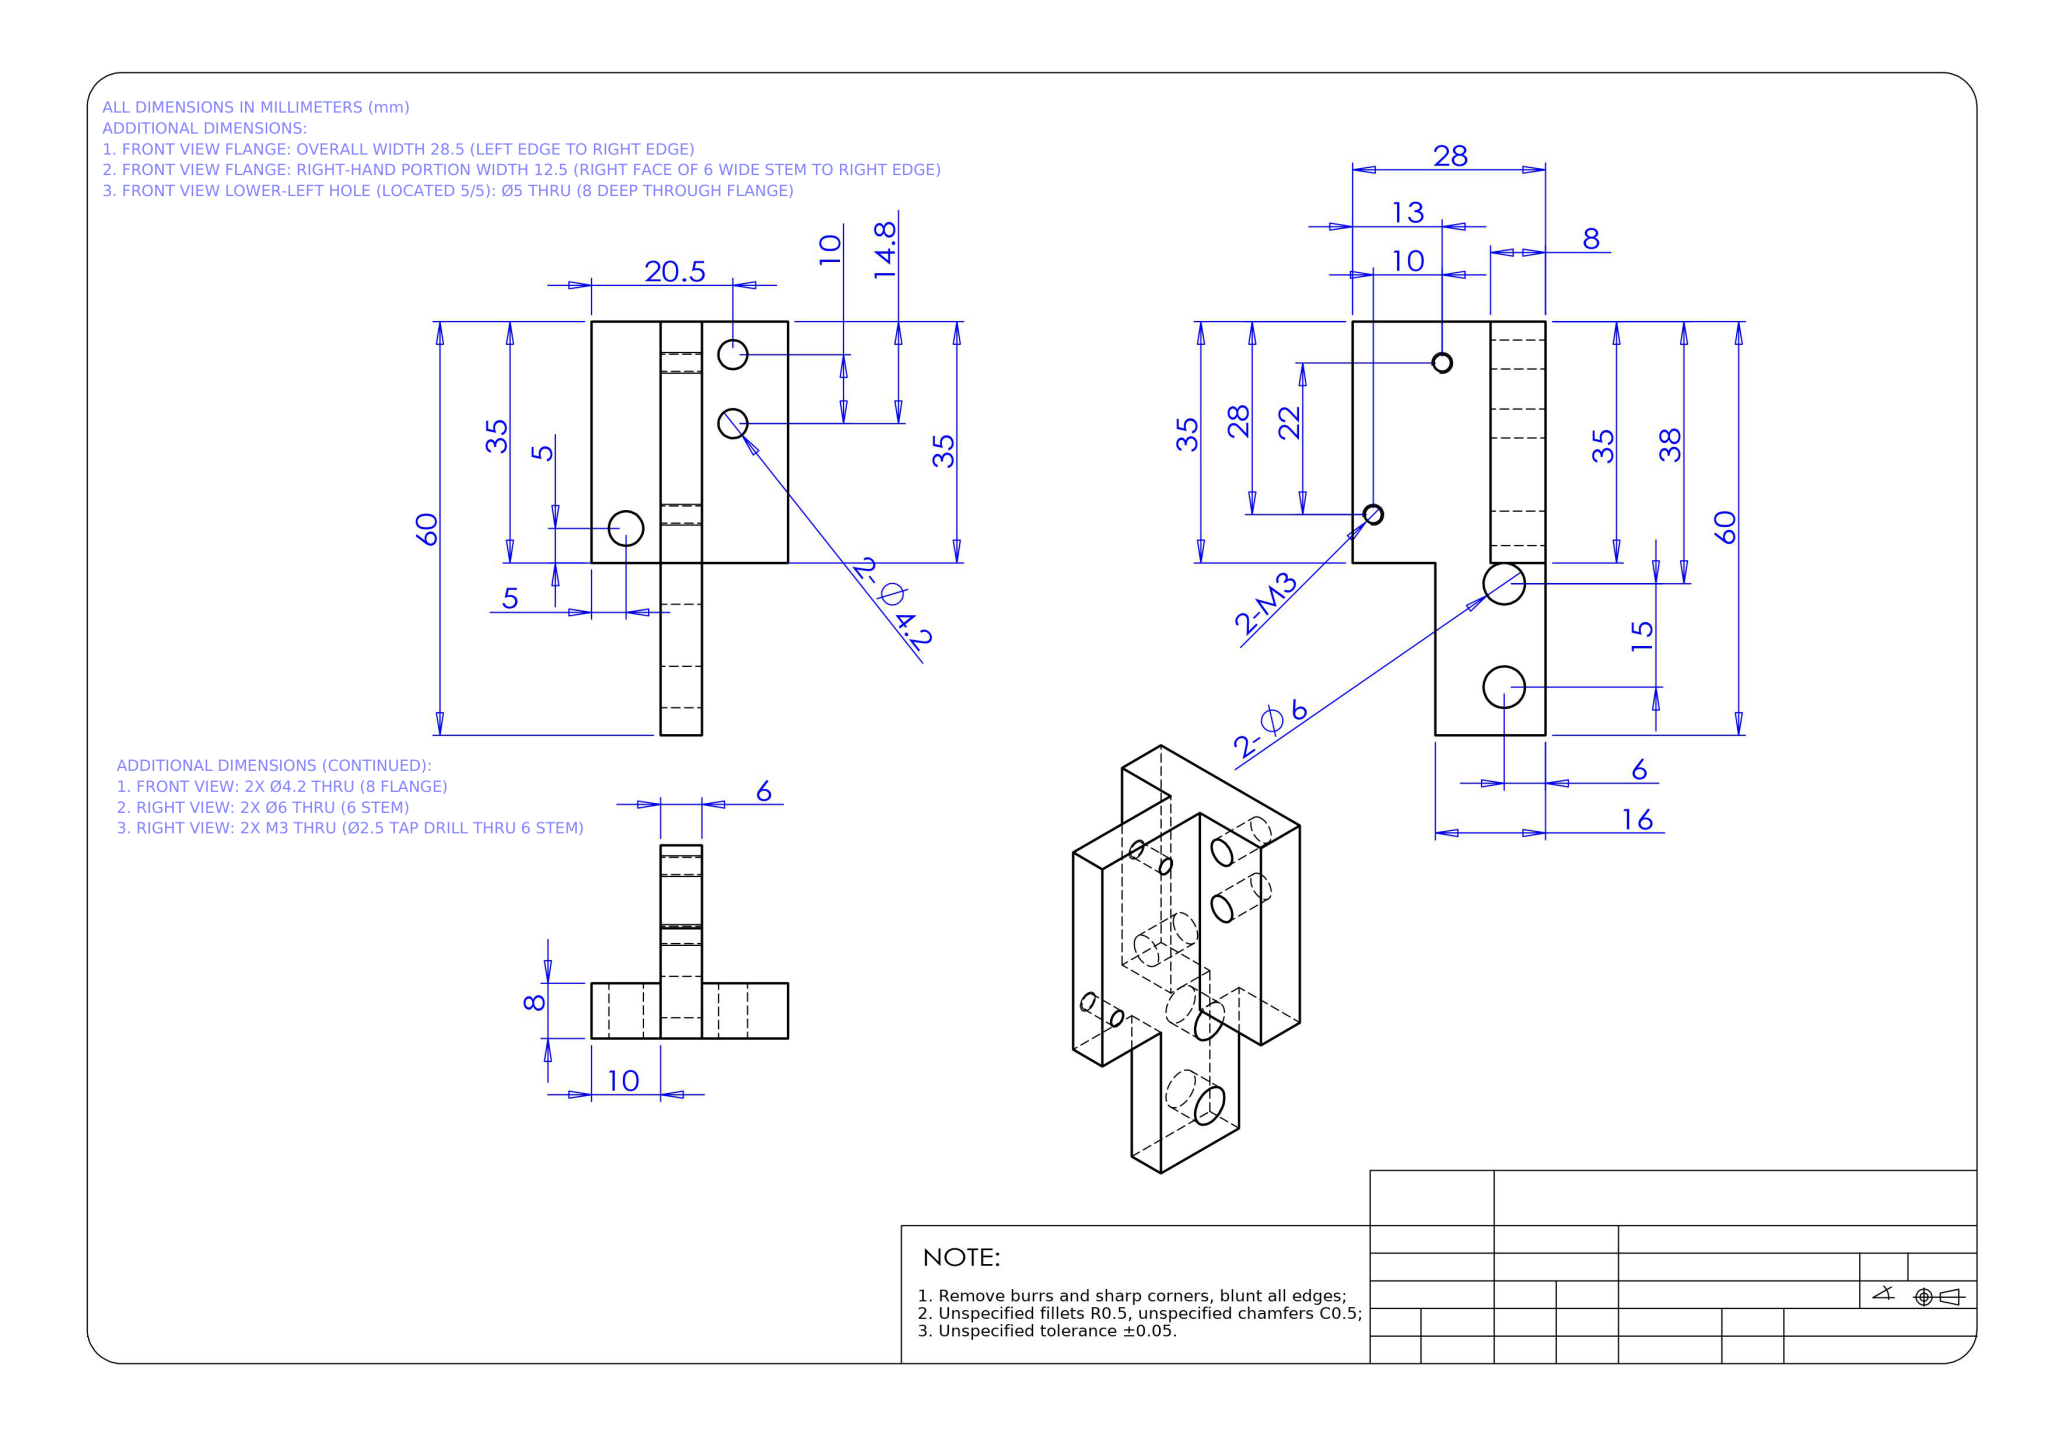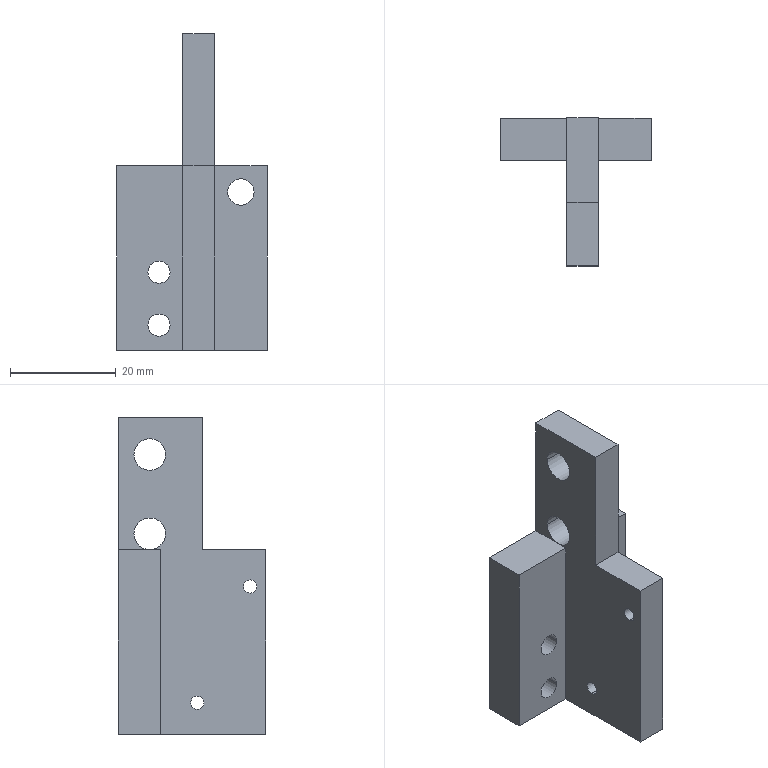Part | NX | mm | 1 solid | 28 faces | box 28.5 x 28 x 60 mm | volume 13803 mm3 | cylinder 14 | plane 14 | commonest cylinder face diameters 6 x4 4.2 x4 2.5 x4 5 x2